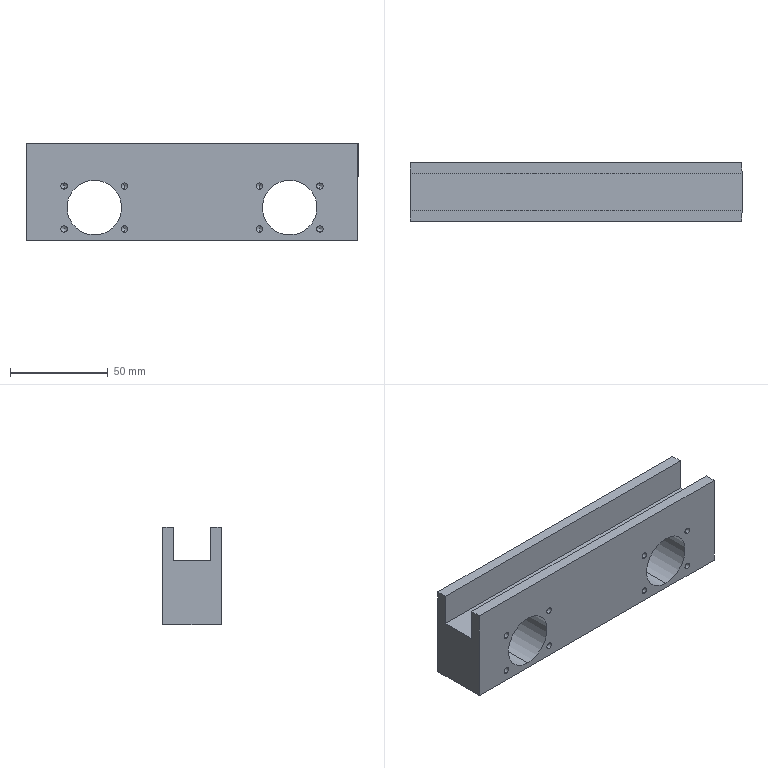Component | SolidWorks | 75-02-14LinearBearingMountingPlate-1 | 1 solid | 62 faces | box 170 x 30 x 50 mm | volume 161721 mm3 | cylinder 28 | cone 24 | plane 10 | commonest cylinder face diameters 3.3 x16 4.2 x8 28 x4 | material A3 Steel
build123d program:
from build123d import *

# Parameters (mm, degrees)
SKETCH1_W             = 170
SKETCH1_H             = 30
BOSS_EXTRUDE1_DEPTH   = 25
SKETCH2_R             = 14
CUT_EXTRUDE1_DEPTH    = 94.541
M4_TAPPED_HOLE1_D     = 3.3
M4_TAPPED_HOLE1_DEPTH = 10.1
M4_TAPPED_HOLE1_TIP   = 0.9914
SKETCH5_W             = 170
SKETCH5_H             = 19
CUT_EXTRUDE2_DEPTH    = 17
M5_TAPPED_HOLE1_D     = 4.2
M5_TAPPED_HOLE1_DEPTH = 12.4
M5_TAPPED_HOLE1_TIP   = 1.262


with BuildPart() as part:
    # Sketch1 → Boss-Extrude1 (new, symmetric)
    with BuildSketch(Plane.XY):
        Rectangle(SKETCH1_W, SKETCH1_H)
    extrude(amount=BOSS_EXTRUDE1_DEPTH, both=True)

    # Sketch2 → Cut-Extrude1 (cut, through all)
    with BuildSketch(Plane(origin=(0, 15, 0), x_dir=(1, 0, 0), z_dir=(0, 1, 0))):
        with Locations(Location((-50, 8, 0), (0, 0, 270))):
            Circle(SKETCH2_R)
        with Locations(Location((50, 8, 0), (0, 0, 270))):
            Circle(SKETCH2_R)
    extrude(amount=-CUT_EXTRUDE1_DEPTH, mode=Mode.SUBTRACT)

    # M4 Tapped Hole1
    with Locations(Plane(origin=(-65.5, 15, 3), x_dir=(0, 0, 1), z_dir=(0, 1, 0))):
        with Locations((0, 0), (0, 31), (-22, 31), (-22, 0), (0, 100), (-22, 100), (0, 131), (-22, 131)):
            Hole(M4_TAPPED_HOLE1_D / 2, depth=M4_TAPPED_HOLE1_DEPTH)
            with Locations((0, 0, -(M4_TAPPED_HOLE1_DEPTH + M4_TAPPED_HOLE1_TIP / 2))):  # 118° drill point
                Cone(0, M4_TAPPED_HOLE1_D / 2, M4_TAPPED_HOLE1_TIP, mode=Mode.SUBTRACT)

    # Sketch5 → Cut-Extrude2 (cut)
    with BuildSketch(Plane.XY.offset(25)):
        Rectangle(SKETCH5_W, SKETCH5_H)
    extrude(amount=-CUT_EXTRUDE2_DEPTH, mode=Mode.SUBTRACT)

    # M5 Tapped Hole1
    with Locations(Plane(origin=(27.5, 10, -25), x_dir=(-1, 0, 0), z_dir=(0, 0, -1))):
        with Locations((0, 0), (55, 0), (55, -20), (0, -20)):
            Hole(M5_TAPPED_HOLE1_D / 2, depth=M5_TAPPED_HOLE1_DEPTH)
            with Locations((0, 0, -(M5_TAPPED_HOLE1_DEPTH + M5_TAPPED_HOLE1_TIP / 2))):  # 118° drill point
                Cone(0, M5_TAPPED_HOLE1_D / 2, M5_TAPPED_HOLE1_TIP, mode=Mode.SUBTRACT)


solid = part.part

# Placed as in the assembly
solid = solid.moved(Location((-17.8, 86.857, 37.75), (0, 0, 180)))